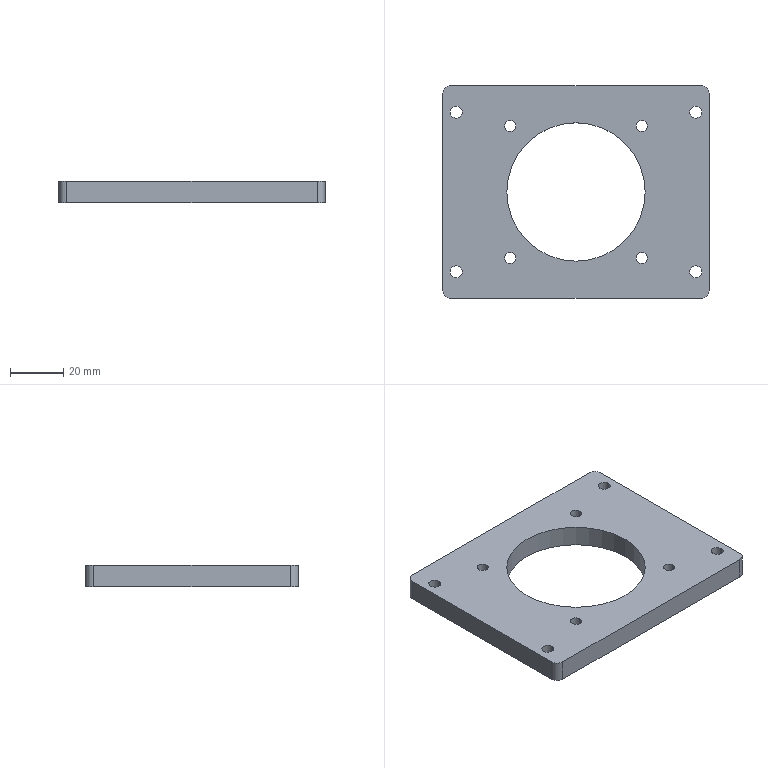CAM job | Mastercam | mm | 8 operations | part box 100 x 80 x 8
1. Facing | 20 - 63 平铣刀
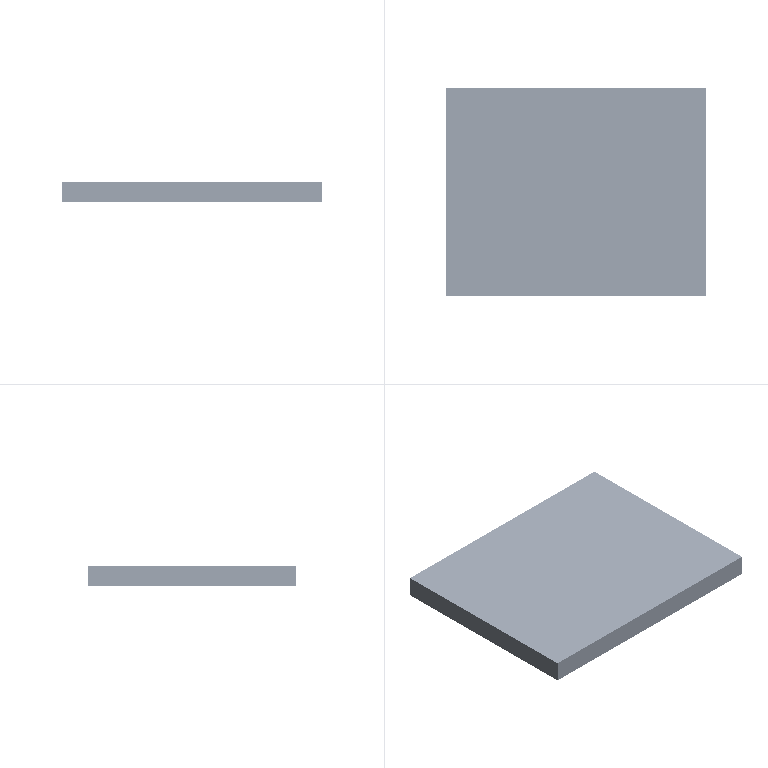2. Contour (Ramp) | 10 - 10 平铣刀
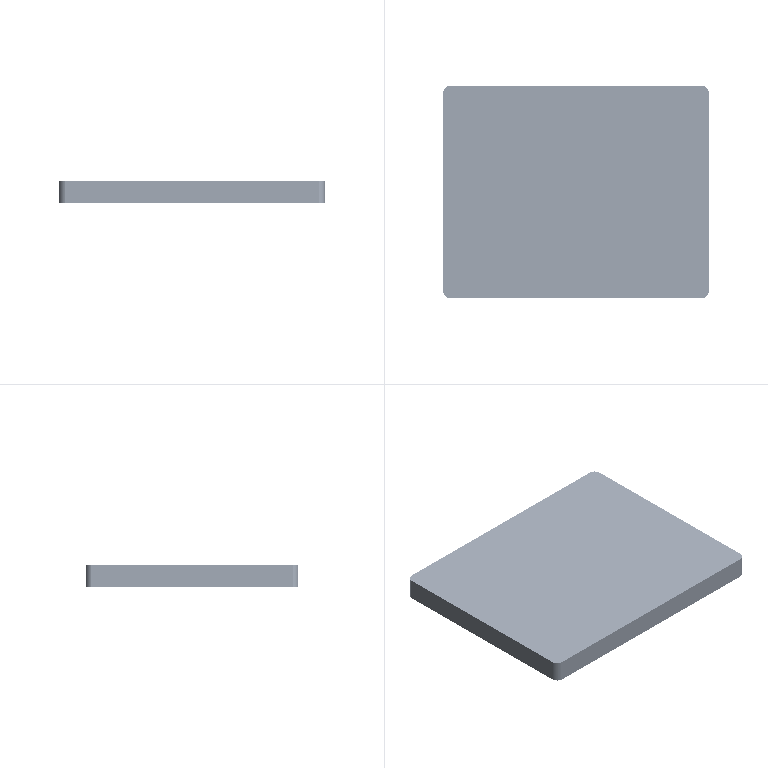3. 2D High Speed (2D Area Mill) | 10 - 10 平铣刀
4. Contour (2D) | 10 - 10 平铣刀
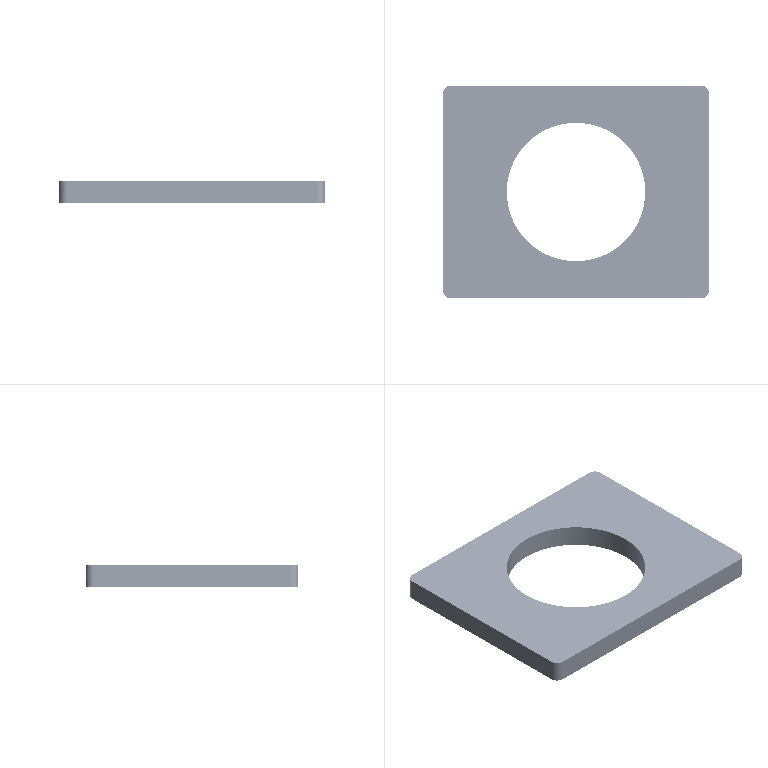5. Drill/Counterbore | 7 - 4 倒角刀
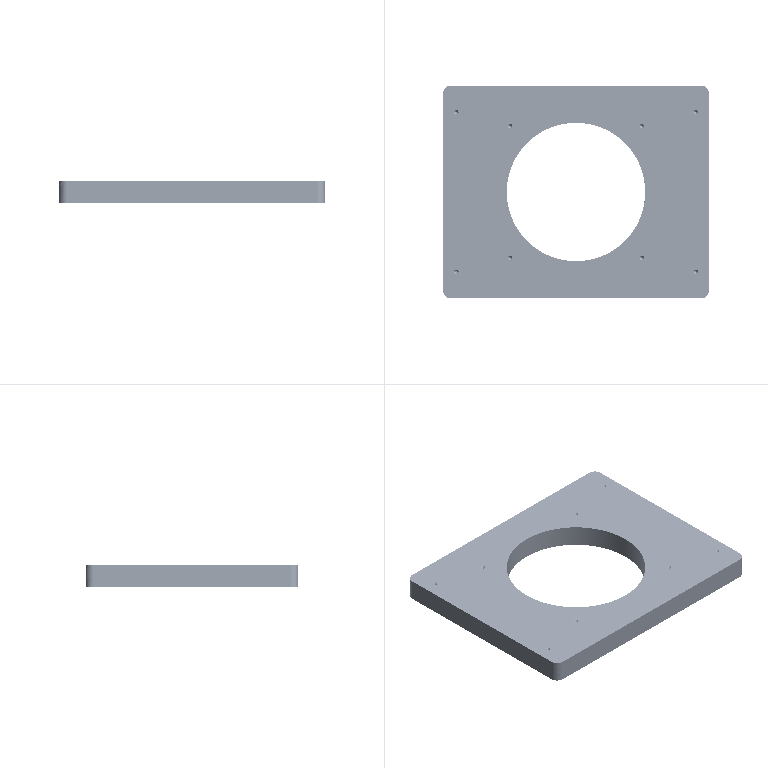6. Contour (2D chamfer) | 7 - 4 倒角刀
7. Facing | 10 - 10 平铣刀
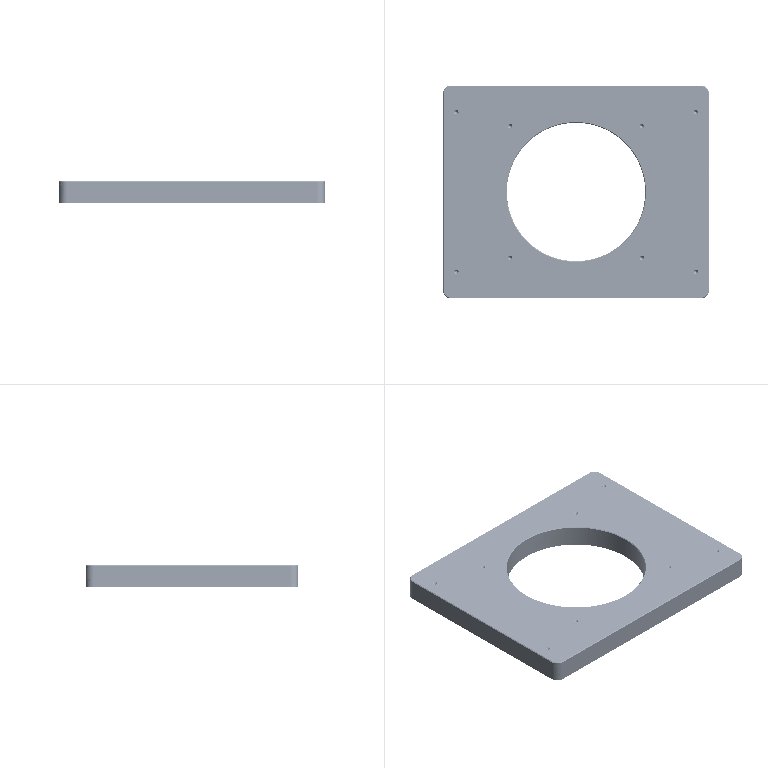8. Contour (2D chamfer) | 7 - 4 倒角刀